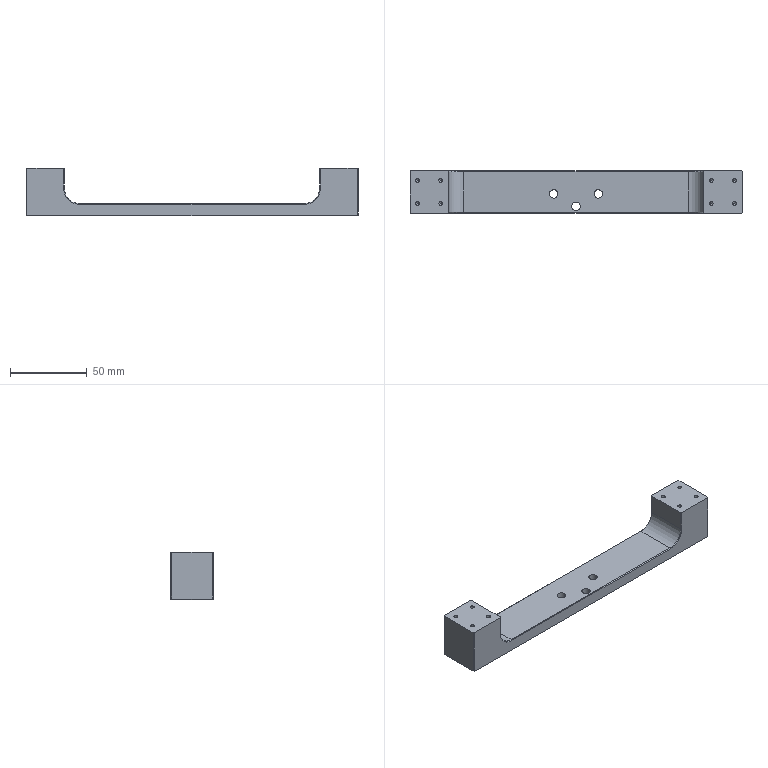Part | SolidWorks | mm | 1 solid | 66 faces | box 216 x 27.5 x 31 mm | volume 79378 mm3 | cylinder 24 | plane 22 | cone 20 | commonest cylinder face diameters 2.5 x16 5.5 x6 20 x2
build123d program:
from build123d import *

# Parameters (mm, degrees)
SKETCH1_W             = 216
SKETCH1_H             = 27.5
BOSS_EXTRUDE1_DEPTH   = 31
SKETCH2_W             = 166
SKETCH2_H             = 46
CUT_EXTRUDE1_DEPTH    = 116.677
M3_TAPPED_HOLE1_D     = 2.5
M3_TAPPED_HOLE1_DEPTH = 7.5
M3_TAPPED_HOLE1_TIP   = 0.7511
M5_CLEARANCE_HOLE1_D  = 5.5
FILLET1_R             = 10
CHAMFER1_SIZE         = 0.5


with BuildPart() as part:
    # Sketch1 → Boss-Extrude1 (new body)
    with BuildSketch(Plane.XY):
        Rectangle(SKETCH1_W, SKETCH1_H)
    extrude(amount=BOSS_EXTRUDE1_DEPTH)

    # Sketch2 → Cut-Extrude1 (cut, through all)
    with BuildSketch(Plane.XZ.offset(13.75)):
        with Locations((0, 31)):
            Rectangle(SKETCH2_W, SKETCH2_H)
    extrude(amount=-CUT_EXTRUDE1_DEPTH, mode=Mode.SUBTRACT)

    # M3 Tapped Hole1
    with Locations(Plane.XY.offset(31)):
        with Locations((-103, 7.5), (-88, 7.5), (-103, -7.5), (-88, -7.5), (88, -7.5), (103, -7.5), (88, 7.5), (103, 7.5)):
            Hole(M3_TAPPED_HOLE1_D / 2, depth=M3_TAPPED_HOLE1_DEPTH)
            with Locations((0, 0, -(M3_TAPPED_HOLE1_DEPTH + M3_TAPPED_HOLE1_TIP / 2))):  # 118° drill point
                Cone(0, M3_TAPPED_HOLE1_D / 2, M3_TAPPED_HOLE1_TIP, mode=Mode.SUBTRACT)

    # M5 Clearance Hole1 (through all)
    with Locations(Plane.XY.offset(8)):
        with Locations((-14.5, -1.25), (0, -9.25), (14.5, -1.25)):
            Hole(M5_CLEARANCE_HOLE1_D / 2)

    # Fillet1
    fillet1_edges = [part.edges().sort_by_distance(p)[0] for p in [
        (83, 0, 8),
        (-83, 0, 8),
    ]]
    fillet(fillet1_edges, radius=FILLET1_R)

    # Chamfer1
    chamfer1_edges = [part.edges().sort_by_distance(p)[0] for p in [
        (-83, 13.75, 24.5),
        (-83, -13.75, 24.5),
        (-108, 0, 0),
        (108, 0, 0),
        (108, -13.75, 15.5),
        (-108, -13.75, 15.5),
        (-108, 13.75, 15.5),
        (108, 13.75, 15.5),
        (83, 13.75, 24.5),
        (83, -13.75, 24.5),
        (0, -13.75, 8),
        (0, 13.75, 8),
        (80.071, -13.75, 10.929),
        (80.071, 13.75, 10.929),
        (-80.071, -13.75, 10.929),
        (-80.071, 13.75, 10.929),
    ]]
    chamfer(chamfer1_edges, length=CHAMFER1_SIZE)


solid = part.part